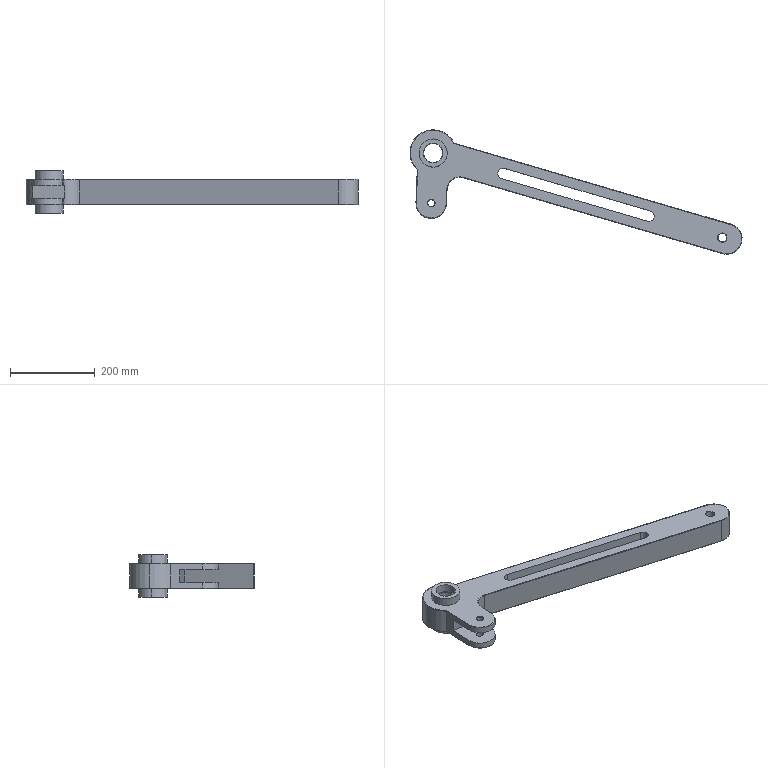Component | SolidWorks | TappingArm-1 | 1 solid | 71 faces | box 781.85 x 292.92 x 100 mm | volume 3234008 mm3 | cylinder 33 | torus 24 | plane 14 | commonest cylinder face diameters 2 x8 46.19 x4 66.486 x4 16 x4 24.909 x3 72 x3 44.19 x2 109.605 x2
build123d program:
from build123d import *

# Parameters (mm, degrees)
SKETCH3_R           = 10
SKETCH3_R_2         = 8
BOSS_EXTRUDE1_DEPTH = 30
SKETCH4_R           = 54.803
BOSS_EXTRUDE2_DEPTH = 60
SKETCH5_R           = 22.095
CUT_EXTRUDE1_DEPTH  = 60
FILLET2_R           = 30
CUT_EXTRUDE2_DEPTH  = 15
FILLET3_R           = 1
CUT_EXTRUDE3_DEPTH  = 230
SKETCH8_R           = 33.243
SKETCH8_R_2         = 23.095
BOSS_EXTRUDE3_DEPTH = 20
BOSS_EXTRUDE4_START = 20
SKETCH9_R           = 33.243
SKETCH9_R_2         = 23.095
BOSS_EXTRUDE4_DEPTH = 20


with BuildPart() as part:
    # Sketch3 → Boss-Extrude1 (new, symmetric)
    # profile 1 of 3: a face of its own
    with BuildSketch(Plane.XY):
        with BuildLine():
            Line((1024.146, -85.48), (312.314, 22.66))
            ThreePointArc((312.314, 22.66), (333.061, 11.806), (342.744, -9.513))
            Line((342.744, -9.513), (347.126, -55.454))
            Line((347.126, -55.454), (1013.332, -156.663))
            ThreePointArc((1013.332, -156.663), (1054.331, -126.478), (1024.146, -85.48))
        make_face()
        with Locations((1007.755, -119.403)):
            Circle(SKETCH3_R, mode=Mode.SUBTRACT)
    # profile 2 of 3: a face of its own
    with BuildSketch(Plane.XY):
        with BuildLine():
            Line((271.069, -16.35), (282.277, -133.849))
            ThreePointArc((282.277, -133.849), (321.533, -166.267), (353.952, -127.012))
            Line((353.952, -127.012), (347.126, -55.454))
            Line((347.126, -55.454), (301.499, -48.523))
            ThreePointArc((301.499, -48.523), (280.752, -37.669), (271.069, -16.35))
        make_face()
        with Locations((318.114, -130.43)):
            Circle(SKETCH3_R_2, mode=Mode.SUBTRACT)
    # profile 3 of 3: a face of its own
    with BuildSketch(Plane.XY):
        with BuildLine():
            ThreePointArc((312.314, 22.66), (282.169, 13.223), (271.069, -16.35))
            ThreePointArc((271.069, -16.35), (280.752, -37.669), (301.499, -48.523))
            Line((301.499, -48.523), (347.126, -55.454))
            Line((347.126, -55.454), (342.744, -9.513))
            ThreePointArc((342.744, -9.513), (333.061, 11.806), (312.314, 22.66))
        make_face()
    extrude(amount=BOSS_EXTRUDE1_DEPTH, both=True)

    # Sketch4 → Boss-Extrude2 (add)
    with BuildSketch(Plane(origin=(0, 0, -30), x_dir=(-1, 0, 0), z_dir=(0, 0, -1))):
        with Locations((-306.906, -12.931)):
            Circle(SKETCH4_R)
    extrude(amount=-BOSS_EXTRUDE2_DEPTH)

    # Sketch5 → Cut-Extrude1 (cut)
    with BuildSketch(Plane(origin=(0, 0, -30), x_dir=(-1, 0, 0), z_dir=(0, 0, -1))):
        with Locations((-306.906, -12.931)):
            Circle(SKETCH5_R)
    extrude(amount=-CUT_EXTRUDE1_DEPTH, mode=Mode.SUBTRACT)

    # Fillet2
    fillet2_edges = [part.edges().sort_by_distance(p)[0] for p in [
        (347.126, -55.454, 0),
    ]]
    fillet(fillet2_edges, radius=FILLET2_R)

    # Sketch6 → Cut-Extrude2 (cut, symmetric)
    with BuildSketch(Plane.XY):
        Polygon((277.184, -80.456), (352.515, -80.456), (365.328, -181.452), (282.324, -185.934), align=None)
    extrude(amount=CUT_EXTRUDE2_DEPTH, both=True, mode=Mode.SUBTRACT)

    # Fillet3
    fillet3_edges = [part.edges().sort_by_distance(p)[0] for p in [
        (310.114, -130.43, -30),
        (997.755, -119.403, -30),
        (1054.331, -126.478, -30),
        (352.365, -110.375, -30),
        (321.533, -166.267, -30),
        (278.635, -95.666, -30),
        (278.635, -95.666, 30),
        (321.533, -166.267, 30),
        (352.365, -110.375, 30),
        (688.655, -34.513, -30),
        (688.655, -34.513, 30),
        (269.249, 26.884, 30),
        (269.249, 26.884, -30),
        (1054.331, -126.478, 30),
        (997.755, -119.403, 30),
        (310.114, -130.43, 30),
        (329.001, -12.931, 30),
        (329.001, -12.931, -30),
        (699.24, -108.947, -30),
        (699.24, -108.947, 30),
        (360.028, -69.095, -30),
        (360.028, -69.095, 30),
    ]]
    fillet(fillet3_edges, radius=FILLET3_R)

    # Sketch7 → Cut-Extrude3 (cut, symmetric)
    with BuildSketch(Plane(origin=(0, 0, -30), x_dir=(-1, 0, 0), z_dir=(0, 0, -1))):
        with BuildLine():
            Line((-831.753, -80.067), (-478.32, -26.374))
            ThreePointArc((-478.32, -26.374), (-464.136, -36.817), (-474.578, -51.001))
            Line((-474.578, -51.001), (-828.011, -104.694))
            ThreePointArc((-828.011, -104.694), (-842.195, -94.251), (-831.753, -80.067))
        make_face()
    extrude(amount=CUT_EXTRUDE3_DEPTH, both=True, mode=Mode.SUBTRACT)

    # Sketch8 → Boss-Extrude3 (add)
    with BuildSketch(Plane.XY.offset(30)):
        with Locations((306.906, -12.931)):
            Circle(SKETCH8_R)
        with Locations((306.906, -12.931)):
            Circle(SKETCH8_R_2, mode=Mode.SUBTRACT)
    extrude(amount=BOSS_EXTRUDE3_DEPTH)

    # Sketch9 → Boss-Extrude4 (add)
    with BuildSketch(Plane(origin=(0, 0, -30), x_dir=(-1, 0, 0), z_dir=(0, 0, -1)).offset(BOSS_EXTRUDE4_START)):
        with Locations(Location((-306.906, -12.931, 0), (0, 0, 180))):
            Circle(SKETCH9_R)
        with Locations(Location((-306.906, -12.931, 0), (0, 0, 180))):
            Circle(SKETCH9_R_2, mode=Mode.SUBTRACT)
    extrude(amount=-BOSS_EXTRUDE4_DEPTH)


solid = part.part

# Placed as in the assembly
solid = solid.moved(Location((4.467, 40.819, 495), (0, 0, -7.665)))